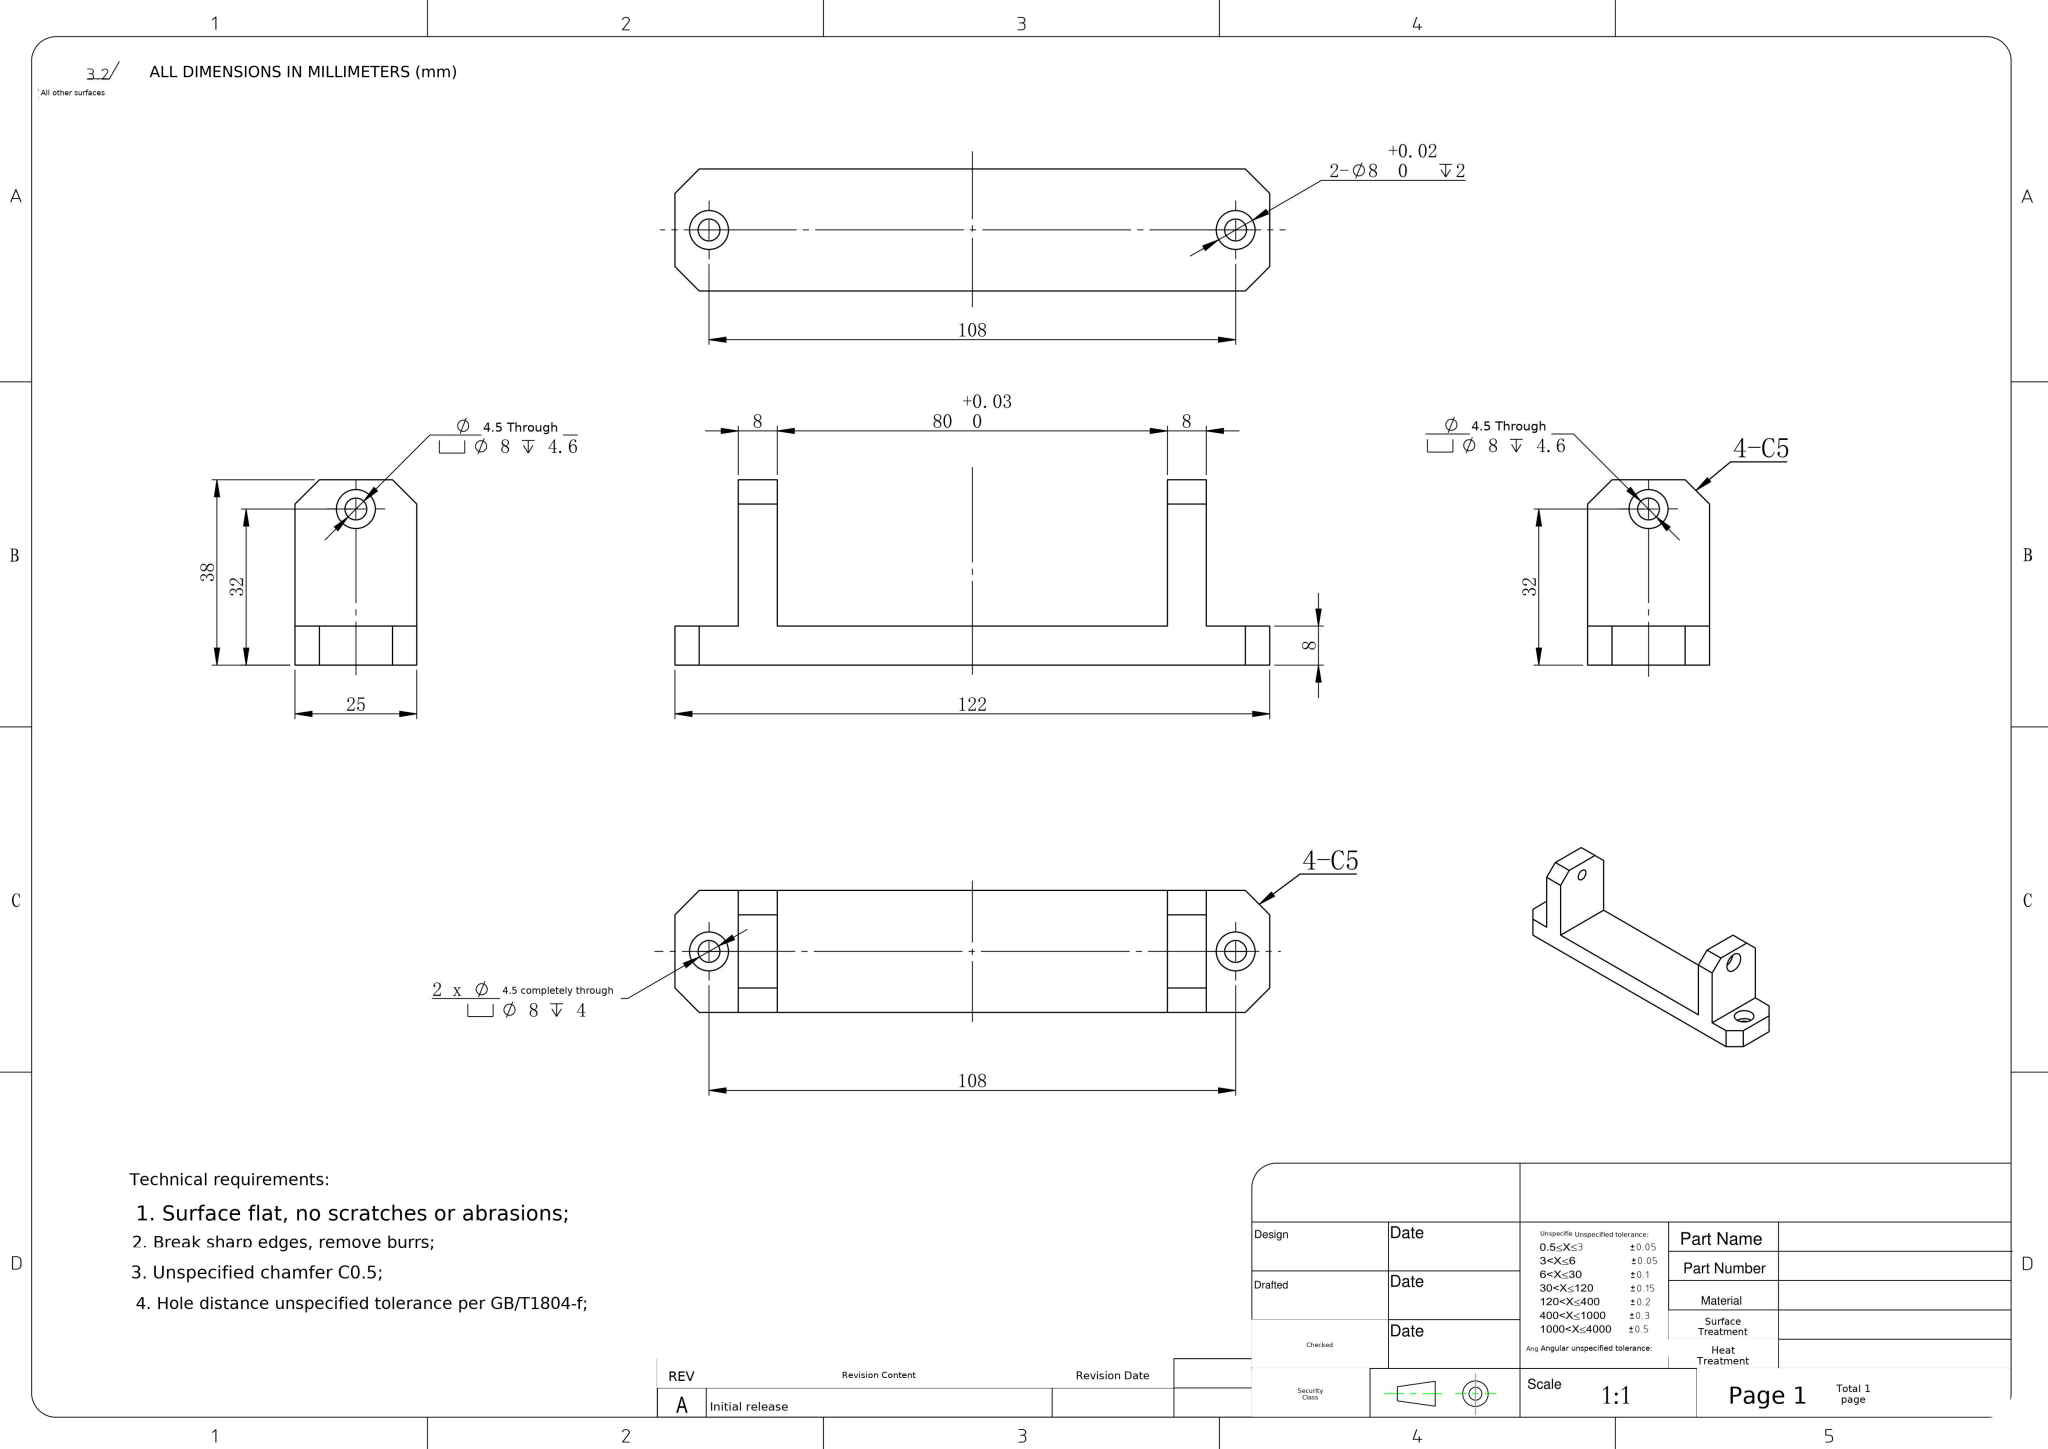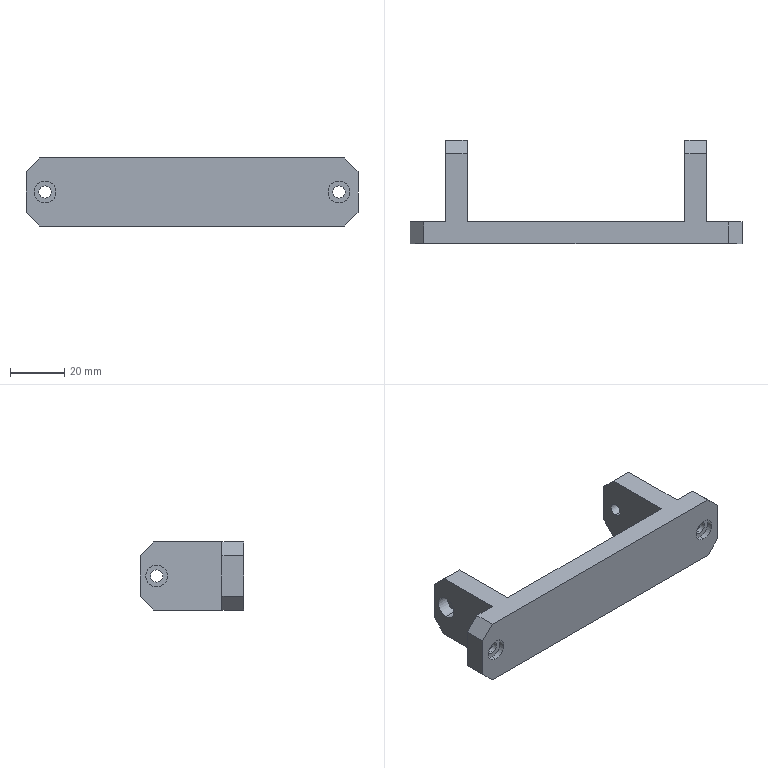Part | NX | mm | 1 solid | 48 faces | box 122 x 38 x 25 mm | volume 34363 mm3 | plane 28 | cylinder 20 | commonest cylinder face diameters 8 x12 4.5 x8